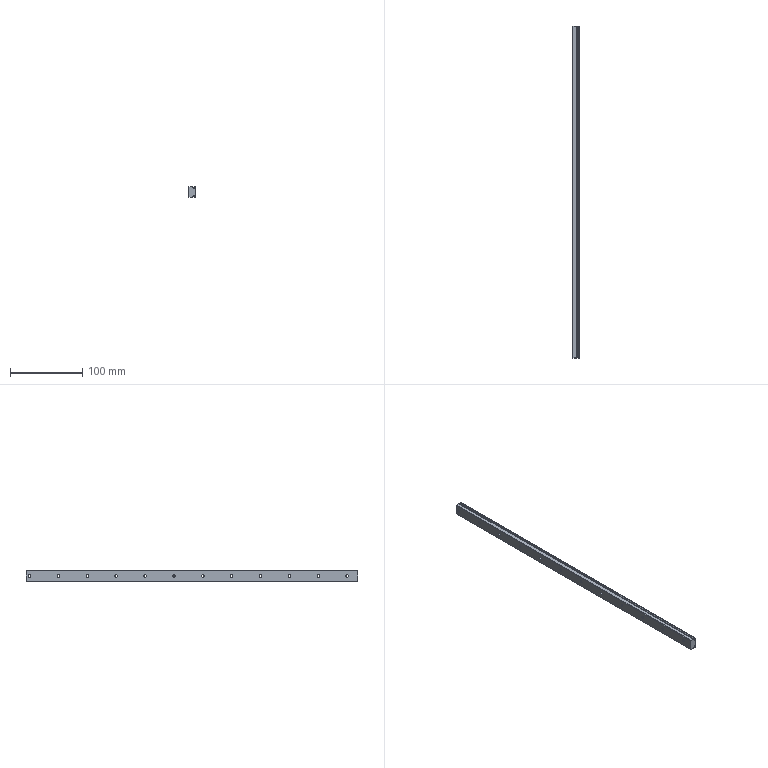Component | SolidWorks | SEBV16-630_2_03-2_r_SEBV16-630-1 | 1 solid | 86 faces | volume 58893 mm3 | cylinder 52 | plane 34 | commonest cylinder face diameters 3.5 x28 6 x24